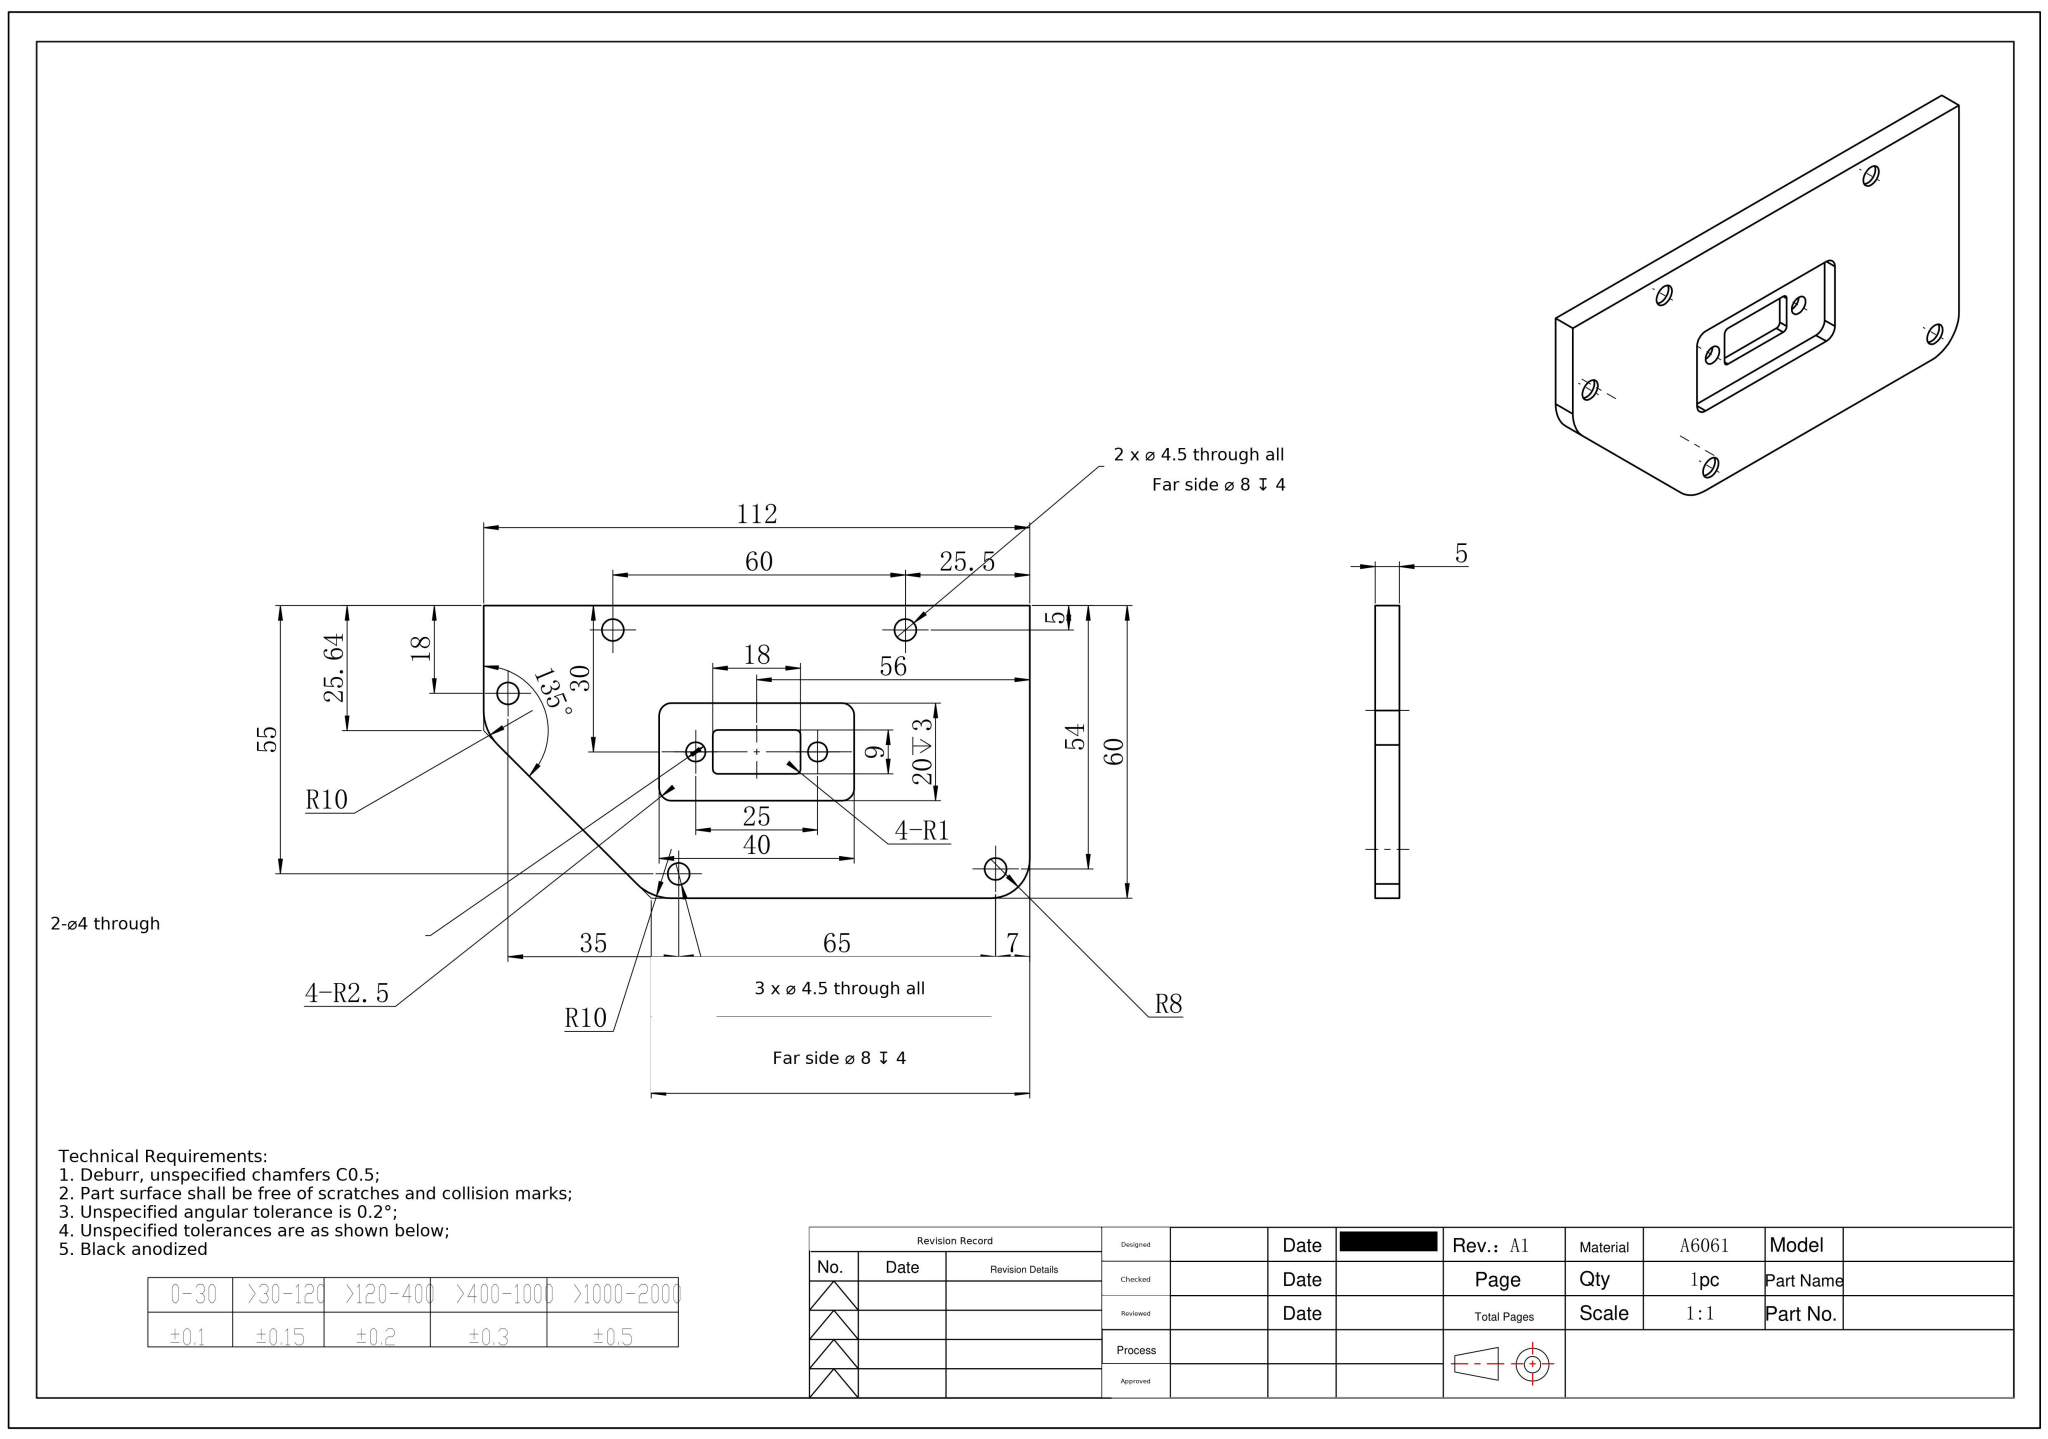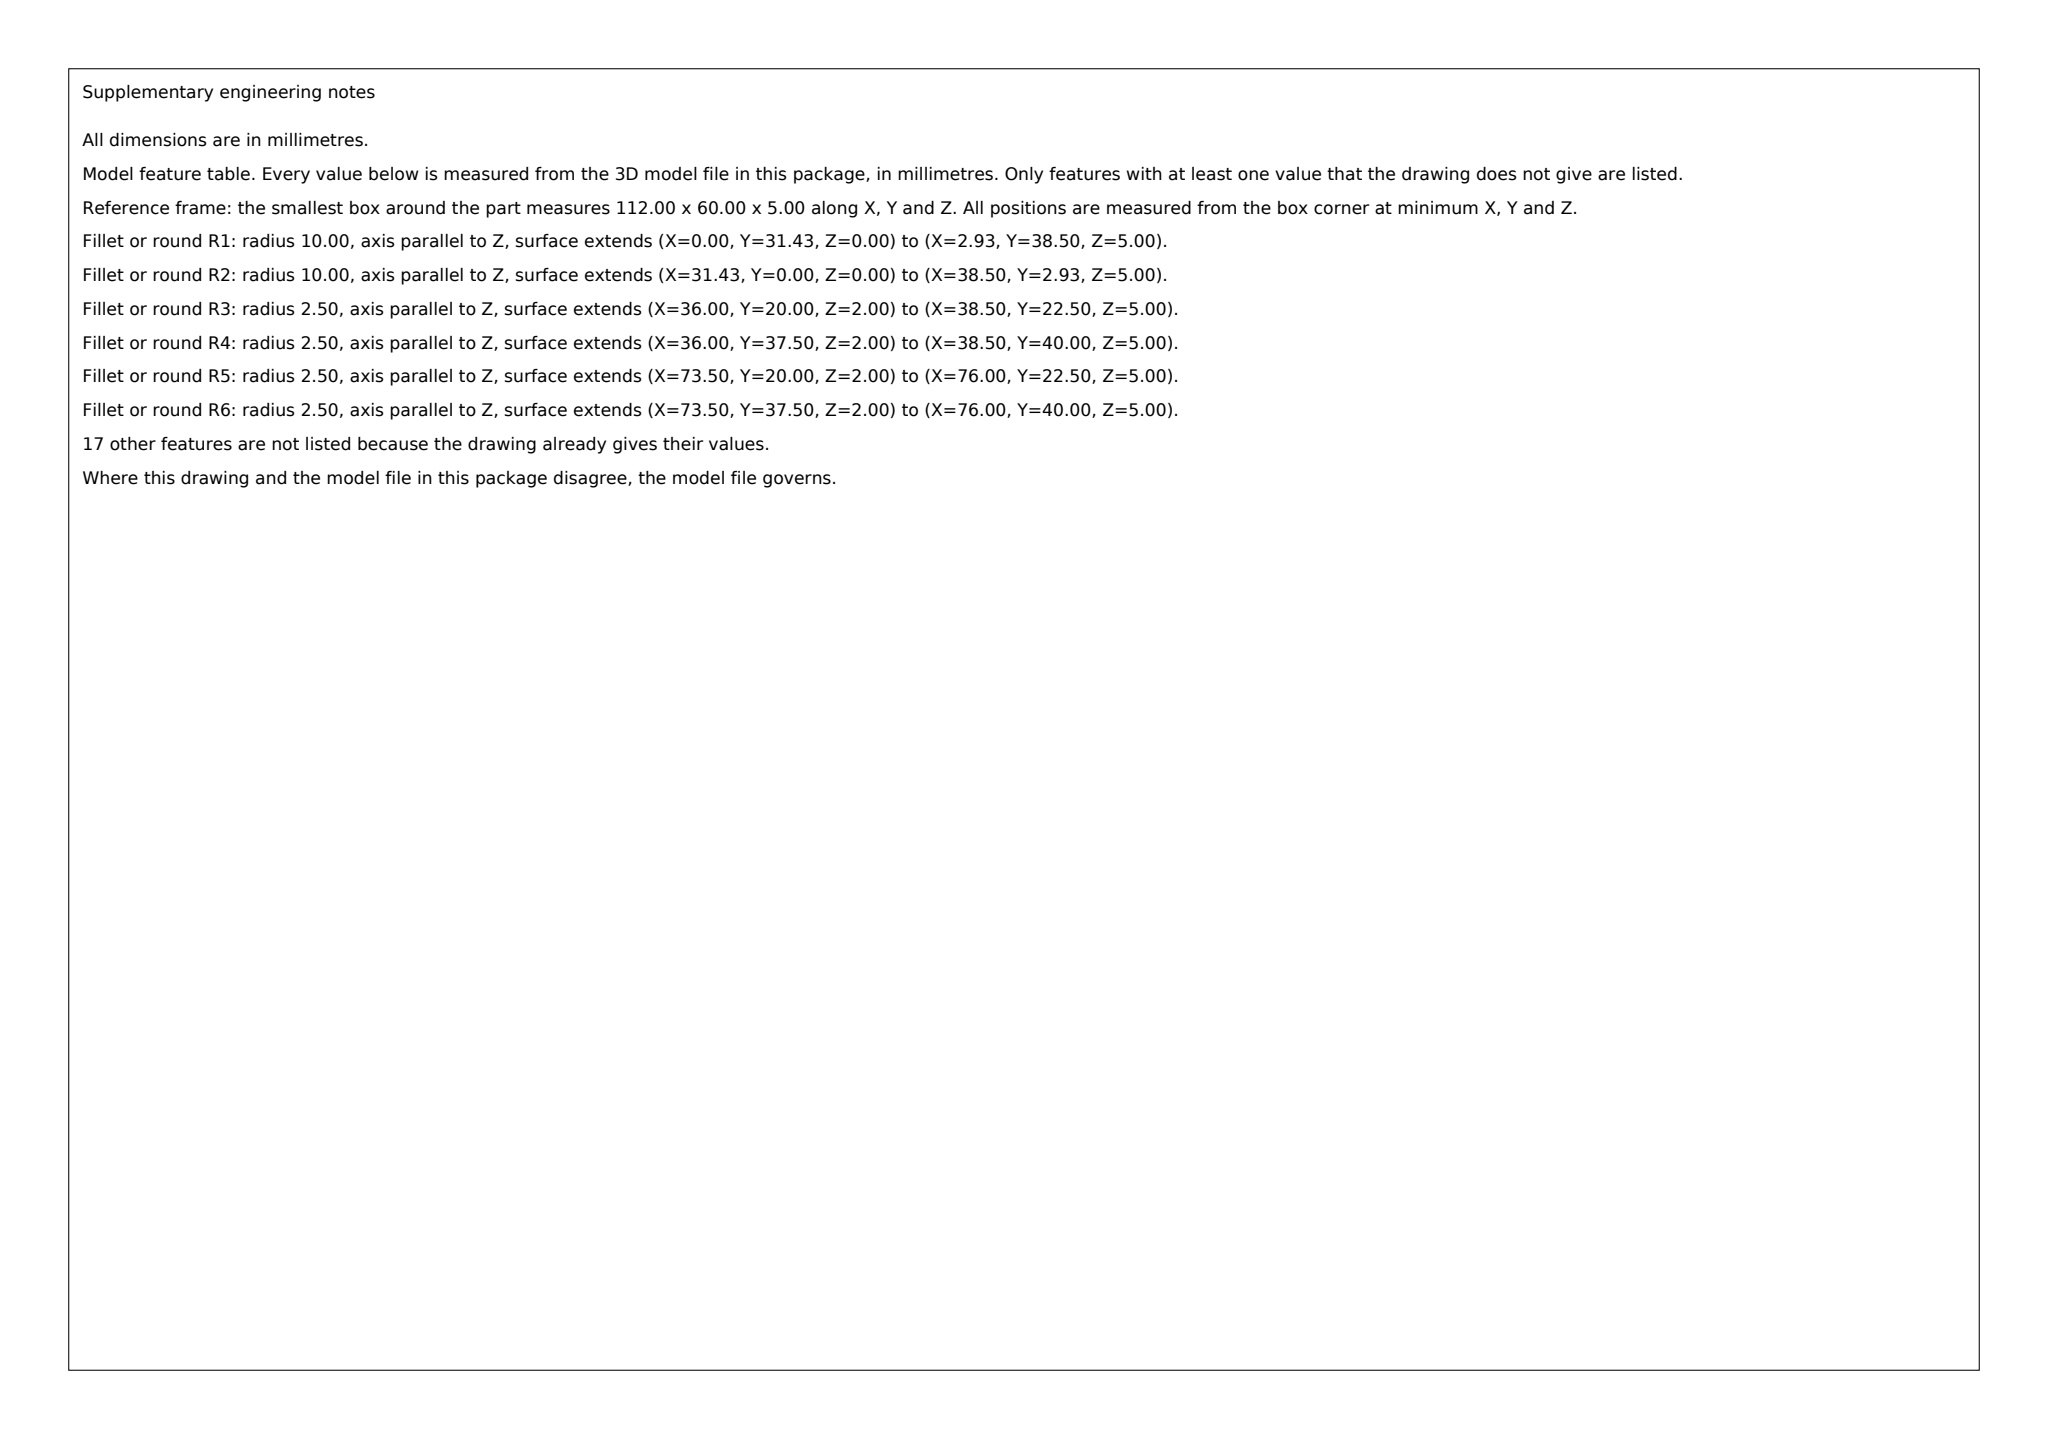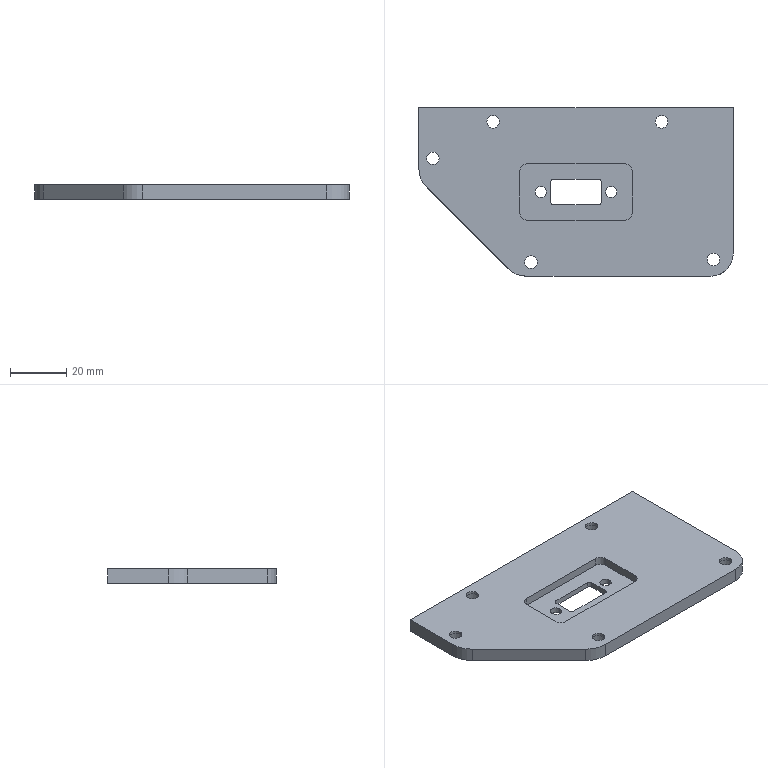Part | SolidWorks | mm | material A6061 | 1 solid | 56 faces | box 112 x 60 x 5 mm | volume 26717 mm3 | cylinder 35 | plane 21 | commonest cylinder face diameters 8 x10 4.5 x10 4 x4 2 x4 5 x4 20 x2 16 x1
build123d program:
from build123d import *

# Parameters (mm, degrees)
SKETCH1_W                                            = 112
SKETCH1_H                                            = 60
BOSS_EXTRUDE1_DEPTH                                  = 2.5
CUT_EXTRUDE1_DEPTH                                   = 10
FILLET1_R                                            = 8
SKETCH3_R                                            = 2
SKETCH3_W                                            = 18
SKETCH3_H                                            = 9
CUT_EXTRUDE2_DEPTH                                   = 10
FILLET2_R                                            = 1
SKETCH4_W                                            = 40
SKETCH4_H                                            = 20
CUT_EXTRUDE3_DEPTH                                   = 3
FILLET3_R                                            = 2.5
HOLE_SIZE_ACCORDING_TO_HEXAGON_SOCKET_HE_D           = 4.5
HOLE_SIZE_ACCORDING_TO_HEXAGON_SOCKET_HE_CBORE_D     = 8
HOLE_SIZE_ACCORDING_TO_HEXAGON_SOCKET_HE_CBORE_DEPTH = 4
HOLE_SIZE_ACCORDING_TO_HEXAGON_SOCKE_2_D             = 4.5
HOLE_SIZE_ACCORDING_TO_HEXAGON_SOCKE_2_CBORE_D       = 8
HOLE_SIZE_ACCORDING_TO_HEXAGON_SOCKE_2_CBORE_DEPTH   = 4


with BuildPart() as part:
    # Sketch1 → Boss-Extrude1 (new, symmetric)
    with BuildSketch(Plane.XY):
        Rectangle(SKETCH1_W, SKETCH1_H)
    extrude(amount=BOSS_EXTRUDE1_DEPTH, both=True)

    # Sketch2 → Cut-Extrude1 (cut)
    with BuildSketch(Plane(origin=(0, 0, -2.5), x_dir=(-1, 0, 0), z_dir=(0, 0, -1))):
        with BuildLine():
            Line((53.071, 1.429), (24.571, -27.071))
            ThreePointArc((24.571, -27.071), (21.327, -29.239), (17.5, -30))
            Line((17.5, -30), (56, -30))
            Line((56, -30), (56, 8.5))
            ThreePointArc((56, 8.5), (55.239, 4.673), (53.071, 1.429))
        make_face()
    extrude(amount=-CUT_EXTRUDE1_DEPTH, mode=Mode.SUBTRACT)

    # Fillet1
    fillet1_edges = [part.edges().sort_by_distance(p)[0] for p in [
        (56, -30, 0),
    ]]
    fillet(fillet1_edges, radius=FILLET1_R)

    # Sketch3 → Cut-Extrude2 (cut)
    with BuildSketch(Plane(origin=(0, 0, -2.5), x_dir=(-1, 0, 0), z_dir=(0, 0, -1))):
        with Locations((-12.5, 0)):
            Circle(SKETCH3_R)
        with Locations(Location((12.5, 0, 0), (0, 0, 180))):
            Circle(SKETCH3_R)
        Rectangle(SKETCH3_W, SKETCH3_H)
    extrude(amount=-CUT_EXTRUDE2_DEPTH, mode=Mode.SUBTRACT)

    # Fillet2
    fillet2_edges = [part.edges().sort_by_distance(p)[0] for p in [
        (-9, 4.5, 0),
        (-9, -4.5, 0),
        (9, -4.5, 0),
        (9, 4.5, 0),
    ]]
    fillet(fillet2_edges, radius=FILLET2_R)

    # Sketch4 → Cut-Extrude3 (cut)
    with BuildSketch(Plane.XY.offset(2.5)):
        Rectangle(SKETCH4_W, SKETCH4_H)
    extrude(amount=-CUT_EXTRUDE3_DEPTH, mode=Mode.SUBTRACT)

    # Fillet3
    fillet3_edges = [part.edges().sort_by_distance(p)[0] for p in [
        (20, 10, 1),
        (20, -10, 1),
        (-20, -10, 1),
        (-20, 10, 1),
    ]]
    fillet(fillet3_edges, radius=FILLET3_R)

    # Hole Size according to Hexagon Socket He (through all)
    with Locations(Plane(origin=(0, 0, -2.5), x_dir=(-1, 0, 0), z_dir=(0, 0, -1))):
        with Locations((-49, -24), (16, -25), (51, 12)):
            CounterBoreHole(HOLE_SIZE_ACCORDING_TO_HEXAGON_SOCKET_HE_D / 2, HOLE_SIZE_ACCORDING_TO_HEXAGON_SOCKET_HE_CBORE_D / 2, HOLE_SIZE_ACCORDING_TO_HEXAGON_SOCKET_HE_CBORE_DEPTH)

    # Hole Size according to Hexagon Socke 2 (through all)
    with Locations(Plane(origin=(0, 0, -2.5), x_dir=(-1, 0, 0), z_dir=(0, 0, -1))):
        with Locations((29.5, 25), (-30.5, 25)):
            CounterBoreHole(HOLE_SIZE_ACCORDING_TO_HEXAGON_SOCKE_2_D / 2, HOLE_SIZE_ACCORDING_TO_HEXAGON_SOCKE_2_CBORE_D / 2, HOLE_SIZE_ACCORDING_TO_HEXAGON_SOCKE_2_CBORE_DEPTH)


solid = part.part